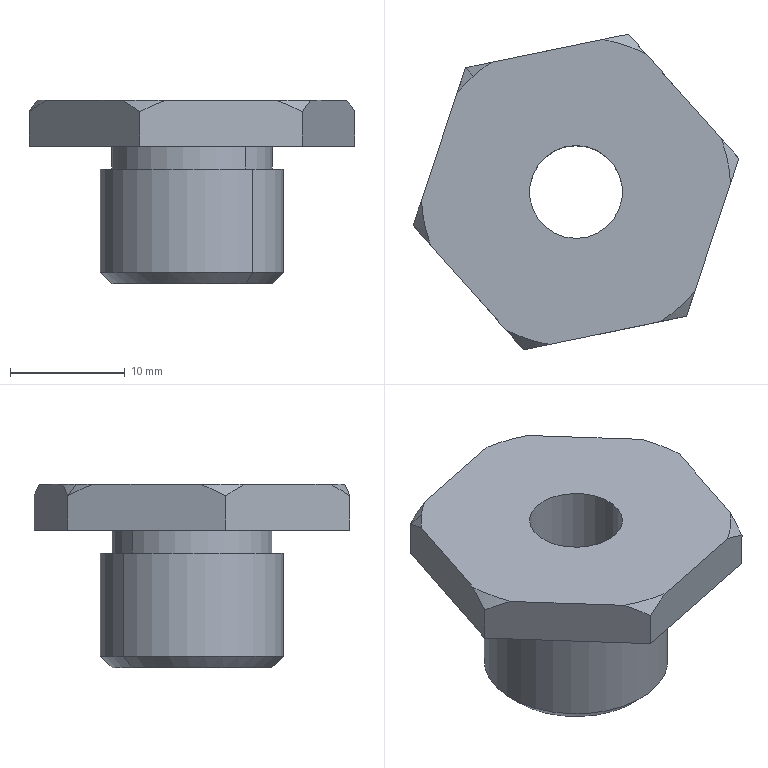Component | SolidWorks | DZ.KX.203-TC1505-20-18-05-93-1 | 1 solid | 25 faces | box 28.4 x 27.52 x 16 mm | volume 3651 mm3 | plane 10 | cone 9 | cylinder 6 | commonest cylinder face diameters 8.1 x2 16 x2 14 x2 | material Plain Carbon Steel
STEP:
#1=COLOUR_RGB('',0.7922,0.8196,0.9333);
#2=FILL_AREA_STYLE_COLOUR('',#1);
#3=FILL_AREA_STYLE('',(#2));
#4=SURFACE_STYLE_FILL_AREA(#3);
#5=SURFACE_SIDE_STYLE('',(#4));
#6=SURFACE_STYLE_USAGE(.BOTH.,#5);
#7=PRESENTATION_STYLE_ASSIGNMENT((#6));
#8=CARTESIAN_POINT('',(11.451,-31.991,4.057));
#9=VERTEX_POINT('',#8);
#10=CARTESIAN_POINT('',(11.817,-32.403,4.057));
#11=VERTEX_POINT('',#10);
#12=CARTESIAN_POINT('',(11.634,-32.197,4.057));
#13=DIRECTION('',(0.,-0.,-1.));
#14=DIRECTION('',(-0.6644,0.7474,-0.));
#15=AXIS2_PLACEMENT_3D('',#12,#13,#14);
#16=CIRCLE('',#15,0.2756);
#17=EDGE_CURVE('',#9,#11,#16,.T.);
#18=ORIENTED_EDGE('',*,*,#17,.F.);
#19=CARTESIAN_POINT('',(11.425,-31.962,4.097));
#20=VERTEX_POINT('',#19);
#21=CARTESIAN_POINT('',(11.451,-31.991,4.057));
#22=DIRECTION('',(-0.4698,0.5285,0.7071));
#23=VECTOR('',#22,39.37);
#24=LINE('',#21,#23);
#25=EDGE_CURVE('',#9,#20,#24,.T.);
#26=ORIENTED_EDGE('',*,*,#25,.T.);
#27=CARTESIAN_POINT('',(11.843,-32.433,4.097));
#28=VERTEX_POINT('',#27);
#29=CARTESIAN_POINT('',(11.634,-32.197,4.097));
#30=DIRECTION('',(-0.,0.,1.));
#31=DIRECTION('',(-0.6644,0.7474,-0.));
#32=AXIS2_PLACEMENT_3D('',#29,#30,#31);
#33=CIRCLE('',#32,0.315);
#34=EDGE_CURVE('',#28,#20,#33,.T.);
#35=ORIENTED_EDGE('',*,*,#34,.F.);
#36=CARTESIAN_POINT('',(11.817,-32.403,4.057));
#37=DIRECTION('',(0.4698,-0.5285,0.7071));
#38=VECTOR('',#37,39.37);
#39=LINE('',#36,#38);
#40=EDGE_CURVE('',#11,#28,#39,.T.);
#41=ORIENTED_EDGE('',*,*,#40,.F.);
#42=EDGE_LOOP('',(#18,#26,#35,#41));
#43=FACE_OUTER_BOUND('',#42,.T.);
#44=CARTESIAN_POINT('',(11.634,-32.197,4.057));
#45=DIRECTION('',(-0.,0.,1.));
#46=DIRECTION('',(0.6644,-0.7474,0.));
#47=AXIS2_PLACEMENT_3D('',#44,#45,#46);
#48=CONICAL_SURFACE('',#47,0.2756,0.7854);
#49=ADVANCED_FACE('',(#43),#48,.T.);
#50=CARTESIAN_POINT('',(11.528,-32.078,4.057));
#51=VERTEX_POINT('',#50);
#52=CARTESIAN_POINT('',(11.74,-32.316,4.057));
#53=VERTEX_POINT('',#52);
#54=CARTESIAN_POINT('',(11.634,-32.197,4.057));
#55=DIRECTION('',(-0.,0.,1.));
#56=DIRECTION('',(0.6644,-0.7474,0.));
#57=AXIS2_PLACEMENT_3D('',#54,#55,#56);
#58=CIRCLE('',#57,0.1594);
#59=EDGE_CURVE('',#51,#53,#58,.T.);
#60=ORIENTED_EDGE('',*,*,#59,.F.);
#61=CARTESIAN_POINT('',(11.528,-32.078,4.687));
#62=VERTEX_POINT('',#61);
#63=CARTESIAN_POINT('',(11.528,-32.078,4.687));
#64=DIRECTION('',(-0.,0.,1.));
#65=VECTOR('',#64,39.37);
#66=LINE('',#63,#65);
#67=EDGE_CURVE('',#51,#62,#66,.T.);
#68=ORIENTED_EDGE('',*,*,#67,.T.);
#69=CARTESIAN_POINT('',(11.74,-32.316,4.687));
#70=VERTEX_POINT('',#69);
#71=CARTESIAN_POINT('',(11.634,-32.197,4.687));
#72=DIRECTION('',(-0.,0.,1.));
#73=DIRECTION('',(0.6644,-0.7474,0.));
#74=AXIS2_PLACEMENT_3D('',#71,#72,#73);
#75=CIRCLE('',#74,0.1594);
#76=EDGE_CURVE('',#62,#70,#75,.T.);
#77=ORIENTED_EDGE('',*,*,#76,.T.);
#78=CARTESIAN_POINT('',(11.74,-32.316,4.687));
#79=DIRECTION('',(-0.,0.,1.));
#80=VECTOR('',#79,39.37);
#81=LINE('',#78,#80);
#82=EDGE_CURVE('',#53,#70,#81,.T.);
#83=ORIENTED_EDGE('',*,*,#82,.F.);
#84=EDGE_LOOP('',(#60,#68,#77,#83));
#85=FACE_OUTER_BOUND('',#84,.T.);
#86=CARTESIAN_POINT('',(11.634,-32.197,4.687));
#87=DIRECTION('',(-0.,0.,1.));
#88=DIRECTION('',(0.6644,-0.7474,0.));
#89=AXIS2_PLACEMENT_3D('',#86,#87,#88);
#90=CYLINDRICAL_SURFACE('',#89,0.1594);
#91=ADVANCED_FACE('',(#85),#90,.F.);
#92=CARTESIAN_POINT('',(11.281,-31.8,4.687));
#93=VERTEX_POINT('',#92);
#94=CARTESIAN_POINT('',(11.226,-31.856,4.687));
#95=VERTEX_POINT('',#94);
#96=CARTESIAN_POINT('',(11.634,-32.197,4.687));
#97=DIRECTION('',(-0.,0.,1.));
#98=DIRECTION('',(-0.6644,0.7474,-0.));
#99=AXIS2_PLACEMENT_3D('',#96,#97,#98);
#100=CIRCLE('',#99,0.5315);
#101=EDGE_CURVE('',#93,#95,#100,.T.);
#102=ORIENTED_EDGE('',*,*,#101,.F.);
#103=CARTESIAN_POINT('',(11.255,-31.77,4.648));
#104=VERTEX_POINT('',#103);
#105=CARTESIAN_POINT('',(11.255,-31.77,4.648));
#106=DIRECTION('',(-0.4698,0.5285,-0.7071));
#107=VECTOR('',#106,39.37);
#108=LINE('',#105,#107);
#109=EDGE_CURVE('',#93,#104,#108,.T.);
#110=ORIENTED_EDGE('',*,*,#109,.T.);
#111=CARTESIAN_POINT('',(11.226,-31.856,4.687));
#112=CARTESIAN_POINT('',(11.231,-31.842,4.682));
#113=CARTESIAN_POINT('',(11.236,-31.827,4.675));
#114=CARTESIAN_POINT('',(11.245,-31.798,4.662));
#115=CARTESIAN_POINT('',(11.25,-31.784,4.655));
#116=CARTESIAN_POINT('',(11.255,-31.77,4.648));
#117=B_SPLINE_CURVE_WITH_KNOTS('',3,(#111,#112,#113,#114,#115,#116),.UNSPECIFIED.,.F.,.F.,(4,2,4),(0.02484,0.02609,0.02734),.UNSPECIFIED.);
#118=EDGE_CURVE('',#95,#104,#117,.T.);
#119=ORIENTED_EDGE('',*,*,#118,.F.);
#120=EDGE_LOOP('',(#102,#110,#119));
#121=FACE_OUTER_BOUND('',#120,.T.);
#122=CARTESIAN_POINT('',(11.634,-32.197,4.648));
#123=DIRECTION('',(0.,-0.,-1.));
#124=DIRECTION('',(-0.6644,0.7474,-0.));
#125=AXIS2_PLACEMENT_3D('',#122,#123,#124);
#126=CONICAL_SURFACE('',#125,0.5709,0.7854);
#127=ADVANCED_FACE('',(#121),#126,.T.);
#128=ORIENTED_EDGE('',*,*,#34,.T.);
#129=CARTESIAN_POINT('',(11.425,-31.962,4.451));
#130=VERTEX_POINT('',#129);
#131=CARTESIAN_POINT('',(11.425,-31.962,4.057));
#132=DIRECTION('',(-0.,0.,1.));
#133=VECTOR('',#132,39.37);
#134=LINE('',#131,#133);
#135=EDGE_CURVE('',#20,#130,#134,.T.);
#136=ORIENTED_EDGE('',*,*,#135,.T.);
#137=CARTESIAN_POINT('',(11.843,-32.433,4.451));
#138=VERTEX_POINT('',#137);
#139=CARTESIAN_POINT('',(11.634,-32.197,4.451));
#140=DIRECTION('',(0.,-0.,-1.));
#141=DIRECTION('',(-0.6644,0.7474,-0.));
#142=AXIS2_PLACEMENT_3D('',#139,#140,#141);
#143=CIRCLE('',#142,0.315);
#144=EDGE_CURVE('',#130,#138,#143,.T.);
#145=ORIENTED_EDGE('',*,*,#144,.T.);
#146=CARTESIAN_POINT('',(11.843,-32.433,4.057));
#147=DIRECTION('',(-0.,0.,1.));
#148=VECTOR('',#147,39.37);
#149=LINE('',#146,#148);
#150=EDGE_CURVE('',#28,#138,#149,.T.);
#151=ORIENTED_EDGE('',*,*,#150,.F.);
#152=EDGE_LOOP('',(#128,#136,#145,#151));
#153=FACE_OUTER_BOUND('',#152,.T.);
#154=CARTESIAN_POINT('',(11.634,-32.197,4.057));
#155=DIRECTION('',(-0.,0.,1.));
#156=DIRECTION('',(0.6644,-0.7474,0.));
#157=AXIS2_PLACEMENT_3D('',#154,#155,#156);
#158=CYLINDRICAL_SURFACE('',#157,0.315);
#159=ADVANCED_FACE('',(#153),#158,.T.);
#160=CARTESIAN_POINT('',(11.451,-31.991,4.451));
#161=VERTEX_POINT('',#160);
#162=CARTESIAN_POINT('',(11.817,-32.403,4.451));
#163=VERTEX_POINT('',#162);
#164=CARTESIAN_POINT('',(11.634,-32.197,4.451));
#165=DIRECTION('',(0.,-0.,-1.));
#166=DIRECTION('',(-0.6644,0.7474,-0.));
#167=AXIS2_PLACEMENT_3D('',#164,#165,#166);
#168=CIRCLE('',#167,0.2756);
#169=EDGE_CURVE('',#161,#163,#168,.T.);
#170=ORIENTED_EDGE('',*,*,#169,.F.);
#171=CARTESIAN_POINT('',(11.451,-31.991,4.53));
#172=VERTEX_POINT('',#171);
#173=CARTESIAN_POINT('',(11.451,-31.991,4.451));
#174=DIRECTION('',(-0.,0.,1.));
#175=VECTOR('',#174,39.37);
#176=LINE('',#173,#175);
#177=EDGE_CURVE('',#161,#172,#176,.T.);
#178=ORIENTED_EDGE('',*,*,#177,.T.);
#179=CARTESIAN_POINT('',(11.817,-32.403,4.53));
#180=VERTEX_POINT('',#179);
#181=CARTESIAN_POINT('',(11.634,-32.197,4.53));
#182=DIRECTION('',(0.,-0.,-1.));
#183=DIRECTION('',(-0.6644,0.7474,-0.));
#184=AXIS2_PLACEMENT_3D('',#181,#182,#183);
#185=CIRCLE('',#184,0.2756);
#186=EDGE_CURVE('',#172,#180,#185,.T.);
#187=ORIENTED_EDGE('',*,*,#186,.T.);
#188=CARTESIAN_POINT('',(11.817,-32.403,4.451));
#189=DIRECTION('',(-0.,0.,1.));
#190=VECTOR('',#189,39.37);
#191=LINE('',#188,#190);
#192=EDGE_CURVE('',#163,#180,#191,.T.);
#193=ORIENTED_EDGE('',*,*,#192,.F.);
#194=EDGE_LOOP('',(#170,#178,#187,#193));
#195=FACE_OUTER_BOUND('',#194,.T.);
#196=CARTESIAN_POINT('',(11.634,-32.197,4.451));
#197=DIRECTION('',(-0.,0.,1.));
#198=DIRECTION('',(0.6644,-0.7474,0.));
#199=AXIS2_PLACEMENT_3D('',#196,#197,#198);
#200=CYLINDRICAL_SURFACE('',#199,0.2756);
#201=ADVANCED_FACE('',(#195),#200,.T.);
#202=CARTESIAN_POINT('',(12.193,-32.082,4.53));
#203=VERTEX_POINT('',#202);
#204=CARTESIAN_POINT('',(12.013,-32.624,4.53));
#205=VERTEX_POINT('',#204);
#206=CARTESIAN_POINT('',(12.193,-32.082,4.53));
#207=DIRECTION('',(-0.315,-0.9491,0.));
#208=VECTOR('',#207,39.37);
#209=LINE('',#206,#208);
#210=EDGE_CURVE('',#203,#205,#209,.T.);
#211=ORIENTED_EDGE('',*,*,#210,.T.);
#212=CARTESIAN_POINT('',(11.454,-32.739,4.53));
#213=VERTEX_POINT('',#212);
#214=CARTESIAN_POINT('',(12.013,-32.624,4.53));
#215=DIRECTION('',(-0.9794,-0.2017,0.));
#216=VECTOR('',#215,39.37);
#217=LINE('',#214,#216);
#218=EDGE_CURVE('',#205,#213,#217,.T.);
#219=ORIENTED_EDGE('',*,*,#218,.T.);
#220=CARTESIAN_POINT('',(11.075,-32.312,4.53));
#221=VERTEX_POINT('',#220);
#222=CARTESIAN_POINT('',(11.454,-32.739,4.53));
#223=DIRECTION('',(-0.6644,0.7474,-0.));
#224=VECTOR('',#223,39.37);
#225=LINE('',#222,#224);
#226=EDGE_CURVE('',#213,#221,#225,.T.);
#227=ORIENTED_EDGE('',*,*,#226,.T.);
#228=CARTESIAN_POINT('',(11.255,-31.77,4.53));
#229=VERTEX_POINT('',#228);
#230=CARTESIAN_POINT('',(11.075,-32.312,4.53));
#231=DIRECTION('',(0.315,0.9491,-0.));
#232=VECTOR('',#231,39.37);
#233=LINE('',#230,#232);
#234=EDGE_CURVE('',#221,#229,#233,.T.);
#235=ORIENTED_EDGE('',*,*,#234,.T.);
#236=CARTESIAN_POINT('',(11.814,-31.655,4.53));
#237=VERTEX_POINT('',#236);
#238=CARTESIAN_POINT('',(11.255,-31.77,4.53));
#239=DIRECTION('',(0.9794,0.2017,-0.));
#240=VECTOR('',#239,39.37);
#241=LINE('',#238,#240);
#242=EDGE_CURVE('',#229,#237,#241,.T.);
#243=ORIENTED_EDGE('',*,*,#242,.T.);
#244=CARTESIAN_POINT('',(11.814,-31.655,4.53));
#245=DIRECTION('',(0.6644,-0.7474,0.));
#246=VECTOR('',#245,39.37);
#247=LINE('',#244,#246);
#248=EDGE_CURVE('',#237,#203,#247,.T.);
#249=ORIENTED_EDGE('',*,*,#248,.T.);
#250=EDGE_LOOP('',(#211,#219,#227,#235,#243,#249));
#251=FACE_OUTER_BOUND('',#250,.T.);
#252=CARTESIAN_POINT('',(11.634,-32.197,4.53));
#253=DIRECTION('',(0.,-0.,-1.));
#254=DIRECTION('',(-0.6644,0.7474,-0.));
#255=AXIS2_PLACEMENT_3D('',#252,#253,#254);
#256=CIRCLE('',#255,0.2756);
#257=EDGE_CURVE('',#180,#172,#256,.T.);
#258=ORIENTED_EDGE('',*,*,#257,.F.);
#259=ORIENTED_EDGE('',*,*,#186,.F.);
#260=EDGE_LOOP('',(#258,#259));
#261=FACE_BOUND('',#260,.T.);
#262=CARTESIAN_POINT('',(11.634,-32.197,4.53));
#263=DIRECTION('',(0.,-0.,-1.));
#264=DIRECTION('',(-0.6644,0.7474,-0.));
#265=AXIS2_PLACEMENT_3D('',#262,#263,#264);
#266=PLANE('',#265);
#267=ADVANCED_FACE('',(#251,#261),#266,.T.);
#268=CARTESIAN_POINT('',(12.193,-32.082,4.648));
#269=VERTEX_POINT('',#268);
#270=CARTESIAN_POINT('',(12.193,-32.082,4.53));
#271=DIRECTION('',(-0.,0.,1.));
#272=VECTOR('',#271,39.37);
#273=LINE('',#270,#272);
#274=EDGE_CURVE('',#203,#269,#273,.T.);
#275=ORIENTED_EDGE('',*,*,#274,.T.);
#276=CARTESIAN_POINT('',(12.165,-32.168,4.687));
#277=VERTEX_POINT('',#276);
#278=CARTESIAN_POINT('',(12.193,-32.082,4.648));
#279=CARTESIAN_POINT('',(12.184,-32.11,4.663));
#280=CARTESIAN_POINT('',(12.174,-32.138,4.676));
#281=CARTESIAN_POINT('',(12.165,-32.168,4.687));
#282=B_SPLINE_CURVE_WITH_KNOTS('',3,(#278,#279,#280,#281),.UNSPECIFIED.,.F.,.F.,(4,4),(0.01221,0.01471),.UNSPECIFIED.);
#283=EDGE_CURVE('',#269,#277,#282,.T.);
#284=ORIENTED_EDGE('',*,*,#283,.T.);
#285=CARTESIAN_POINT('',(12.042,-32.538,4.687));
#286=VERTEX_POINT('',#285);
#287=CARTESIAN_POINT('',(12.193,-32.082,4.687));
#288=DIRECTION('',(-0.315,-0.9491,0.));
#289=VECTOR('',#288,39.37);
#290=LINE('',#287,#289);
#291=EDGE_CURVE('',#277,#286,#290,.T.);
#292=ORIENTED_EDGE('',*,*,#291,.T.);
#293=CARTESIAN_POINT('',(12.013,-32.624,4.648));
#294=VERTEX_POINT('',#293);
#295=CARTESIAN_POINT('',(12.042,-32.538,4.687));
#296=CARTESIAN_POINT('',(12.037,-32.553,4.682));
#297=CARTESIAN_POINT('',(12.032,-32.567,4.675));
#298=CARTESIAN_POINT('',(12.022,-32.596,4.662));
#299=CARTESIAN_POINT('',(12.018,-32.61,4.655));
#300=CARTESIAN_POINT('',(12.013,-32.624,4.648));
#301=B_SPLINE_CURVE_WITH_KNOTS('',3,(#295,#296,#297,#298,#299,#300),.UNSPECIFIED.,.F.,.F.,(4,2,4),(0.02484,0.02609,0.02734),.UNSPECIFIED.);
#302=EDGE_CURVE('',#286,#294,#301,.T.);
#303=ORIENTED_EDGE('',*,*,#302,.T.);
#304=CARTESIAN_POINT('',(12.013,-32.624,4.53));
#305=DIRECTION('',(-0.,0.,1.));
#306=VECTOR('',#305,39.37);
#307=LINE('',#304,#306);
#308=EDGE_CURVE('',#205,#294,#307,.T.);
#309=ORIENTED_EDGE('',*,*,#308,.F.);
#310=ORIENTED_EDGE('',*,*,#210,.F.);
#311=EDGE_LOOP('',(#275,#284,#292,#303,#309,#310));
#312=FACE_OUTER_BOUND('',#311,.T.);
#313=CARTESIAN_POINT('',(12.193,-32.082,4.53));
#314=DIRECTION('',(-0.9491,0.315,-0.));
#315=DIRECTION('',(0.315,0.9491,-0.));
#316=AXIS2_PLACEMENT_3D('',#313,#314,#315);
#317=PLANE('',#316);
#318=ADVANCED_FACE('',(#312),#317,.F.);
#319=ORIENTED_EDGE('',*,*,#308,.T.);
#320=CARTESIAN_POINT('',(11.925,-32.642,4.687));
#321=VERTEX_POINT('',#320);
#322=CARTESIAN_POINT('',(12.013,-32.624,4.648));
#323=CARTESIAN_POINT('',(11.984,-32.63,4.663));
#324=CARTESIAN_POINT('',(11.955,-32.636,4.676));
#325=CARTESIAN_POINT('',(11.925,-32.642,4.687));
#326=B_SPLINE_CURVE_WITH_KNOTS('',3,(#322,#323,#324,#325),.UNSPECIFIED.,.F.,.F.,(4,4),(0.01221,0.01471),.UNSPECIFIED.);
#327=EDGE_CURVE('',#294,#321,#326,.T.);
#328=ORIENTED_EDGE('',*,*,#327,.T.);
#329=CARTESIAN_POINT('',(11.542,-32.721,4.687));
#330=VERTEX_POINT('',#329);
#331=CARTESIAN_POINT('',(12.013,-32.624,4.687));
#332=DIRECTION('',(-0.9794,-0.2017,0.));
#333=VECTOR('',#332,39.37);
#334=LINE('',#331,#333);
#335=EDGE_CURVE('',#321,#330,#334,.T.);
#336=ORIENTED_EDGE('',*,*,#335,.T.);
#337=CARTESIAN_POINT('',(11.454,-32.739,4.648));
#338=VERTEX_POINT('',#337);
#339=CARTESIAN_POINT('',(11.542,-32.721,4.687));
#340=CARTESIAN_POINT('',(11.527,-32.724,4.682));
#341=CARTESIAN_POINT('',(11.512,-32.727,4.675));
#342=CARTESIAN_POINT('',(11.483,-32.733,4.662));
#343=CARTESIAN_POINT('',(11.468,-32.736,4.655));
#344=CARTESIAN_POINT('',(11.454,-32.739,4.648));
#345=B_SPLINE_CURVE_WITH_KNOTS('',3,(#339,#340,#341,#342,#343,#344),.UNSPECIFIED.,.F.,.F.,(4,2,4),(0.02484,0.02609,0.02734),.UNSPECIFIED.);
#346=EDGE_CURVE('',#330,#338,#345,.T.);
#347=ORIENTED_EDGE('',*,*,#346,.T.);
#348=CARTESIAN_POINT('',(11.454,-32.739,4.53));
#349=DIRECTION('',(-0.,0.,1.));
#350=VECTOR('',#349,39.37);
#351=LINE('',#348,#350);
#352=EDGE_CURVE('',#213,#338,#351,.T.);
#353=ORIENTED_EDGE('',*,*,#352,.F.);
#354=ORIENTED_EDGE('',*,*,#218,.F.);
#355=EDGE_LOOP('',(#319,#328,#336,#347,#353,#354));
#356=FACE_OUTER_BOUND('',#355,.T.);
#357=CARTESIAN_POINT('',(12.013,-32.624,4.53));
#358=DIRECTION('',(-0.2017,0.9794,-0.));
#359=DIRECTION('',(0.9794,0.2017,-0.));
#360=AXIS2_PLACEMENT_3D('',#357,#358,#359);
#361=PLANE('',#360);
#362=ADVANCED_FACE('',(#356),#361,.F.);
#363=ORIENTED_EDGE('',*,*,#352,.T.);
#364=CARTESIAN_POINT('',(11.394,-32.671,4.687));
#365=VERTEX_POINT('',#364);
#366=CARTESIAN_POINT('',(11.454,-32.739,4.648));
#367=CARTESIAN_POINT('',(11.435,-32.717,4.663));
#368=CARTESIAN_POINT('',(11.414,-32.694,4.676));
#369=CARTESIAN_POINT('',(11.394,-32.671,4.687));
#370=B_SPLINE_CURVE_WITH_KNOTS('',3,(#366,#367,#368,#369),.UNSPECIFIED.,.F.,.F.,(4,4),(0.01048,0.01297),.UNSPECIFIED.);
#371=EDGE_CURVE('',#338,#365,#370,.T.);
#372=ORIENTED_EDGE('',*,*,#371,.T.);
#373=CARTESIAN_POINT('',(11.135,-32.38,4.687));
#374=VERTEX_POINT('',#373);
#375=CARTESIAN_POINT('',(11.454,-32.739,4.687));
#376=DIRECTION('',(-0.6644,0.7474,-0.));
#377=VECTOR('',#376,39.37);
#378=LINE('',#375,#377);
#379=EDGE_CURVE('',#365,#374,#378,.T.);
#380=ORIENTED_EDGE('',*,*,#379,.T.);
#381=CARTESIAN_POINT('',(11.075,-32.312,4.648));
#382=VERTEX_POINT('',#381);
#383=CARTESIAN_POINT('',(11.135,-32.38,4.687));
#384=CARTESIAN_POINT('',(11.114,-32.357,4.676));
#385=CARTESIAN_POINT('',(11.094,-32.334,4.663));
#386=CARTESIAN_POINT('',(11.075,-32.312,4.648));
#387=B_SPLINE_CURVE_WITH_KNOTS('',3,(#383,#384,#385,#386),.UNSPECIFIED.,.F.,.F.,(4,4),(0.02308,0.02558),.UNSPECIFIED.);
#388=EDGE_CURVE('',#374,#382,#387,.T.);
#389=ORIENTED_EDGE('',*,*,#388,.T.);
#390=CARTESIAN_POINT('',(11.075,-32.312,4.53));
#391=DIRECTION('',(-0.,0.,1.));
#392=VECTOR('',#391,39.37);
#393=LINE('',#390,#392);
#394=EDGE_CURVE('',#221,#382,#393,.T.);
#395=ORIENTED_EDGE('',*,*,#394,.F.);
#396=ORIENTED_EDGE('',*,*,#226,.F.);
#397=EDGE_LOOP('',(#363,#372,#380,#389,#395,#396));
#398=FACE_OUTER_BOUND('',#397,.T.);
#399=CARTESIAN_POINT('',(11.454,-32.739,4.53));
#400=DIRECTION('',(0.7474,0.6644,-0.));
#401=DIRECTION('',(0.6644,-0.7474,0.));
#402=AXIS2_PLACEMENT_3D('',#399,#400,#401);
#403=PLANE('',#402);
#404=ADVANCED_FACE('',(#398),#403,.F.);
#405=ORIENTED_EDGE('',*,*,#394,.T.);
#406=CARTESIAN_POINT('',(11.103,-32.227,4.687));
#407=VERTEX_POINT('',#406);
#408=CARTESIAN_POINT('',(11.075,-32.312,4.648));
#409=CARTESIAN_POINT('',(11.084,-32.284,4.663));
#410=CARTESIAN_POINT('',(11.093,-32.256,4.676));
#411=CARTESIAN_POINT('',(11.103,-32.227,4.687));
#412=B_SPLINE_CURVE_WITH_KNOTS('',3,(#408,#409,#410,#411),.UNSPECIFIED.,.F.,.F.,(4,4),(0.01221,0.01471),.UNSPECIFIED.);
#413=EDGE_CURVE('',#382,#407,#412,.T.);
#414=ORIENTED_EDGE('',*,*,#413,.T.);
#415=CARTESIAN_POINT('',(11.075,-32.312,4.687));
#416=DIRECTION('',(0.315,0.9491,-0.));
#417=VECTOR('',#416,39.37);
#418=LINE('',#415,#417);
#419=EDGE_CURVE('',#407,#95,#418,.T.);
#420=ORIENTED_EDGE('',*,*,#419,.T.);
#421=ORIENTED_EDGE('',*,*,#118,.T.);
#422=CARTESIAN_POINT('',(11.255,-31.77,4.53));
#423=DIRECTION('',(-0.,0.,1.));
#424=VECTOR('',#423,39.37);
#425=LINE('',#422,#424);
#426=EDGE_CURVE('',#229,#104,#425,.T.);
#427=ORIENTED_EDGE('',*,*,#426,.F.);
#428=ORIENTED_EDGE('',*,*,#234,.F.);
#429=EDGE_LOOP('',(#405,#414,#420,#421,#427,#428));
#430=FACE_OUTER_BOUND('',#429,.T.);
#431=CARTESIAN_POINT('',(11.075,-32.312,4.53));
#432=DIRECTION('',(0.9491,-0.315,0.));
#433=DIRECTION('',(-0.315,-0.9491,0.));
#434=AXIS2_PLACEMENT_3D('',#431,#432,#433);
#435=PLANE('',#434);
#436=ADVANCED_FACE('',(#430),#435,.F.);
#437=ORIENTED_EDGE('',*,*,#426,.T.);
#438=CARTESIAN_POINT('',(11.343,-31.752,4.687));
#439=VERTEX_POINT('',#438);
#440=CARTESIAN_POINT('',(11.255,-31.77,4.648));
#441=CARTESIAN_POINT('',(11.283,-31.765,4.663));
#442=CARTESIAN_POINT('',(11.313,-31.758,4.676));
#443=CARTESIAN_POINT('',(11.343,-31.752,4.687));
#444=B_SPLINE_CURVE_WITH_KNOTS('',3,(#440,#441,#442,#443),.UNSPECIFIED.,.F.,.F.,(4,4),(0.01221,0.01471),.UNSPECIFIED.);
#445=EDGE_CURVE('',#104,#439,#444,.T.);
#446=ORIENTED_EDGE('',*,*,#445,.T.);
#447=CARTESIAN_POINT('',(11.725,-31.674,4.687));
#448=VERTEX_POINT('',#447);
#449=CARTESIAN_POINT('',(11.255,-31.77,4.687));
#450=DIRECTION('',(0.9794,0.2017,-0.));
#451=VECTOR('',#450,39.37);
#452=LINE('',#449,#451);
#453=EDGE_CURVE('',#439,#448,#452,.T.);
#454=ORIENTED_EDGE('',*,*,#453,.T.);
#455=CARTESIAN_POINT('',(11.814,-31.655,4.648));
#456=VERTEX_POINT('',#455);
#457=CARTESIAN_POINT('',(11.725,-31.674,4.687));
#458=CARTESIAN_POINT('',(11.74,-31.67,4.682));
#459=CARTESIAN_POINT('',(11.755,-31.667,4.675));
#460=CARTESIAN_POINT('',(11.785,-31.661,4.662));
#461=CARTESIAN_POINT('',(11.799,-31.658,4.655));
#462=CARTESIAN_POINT('',(11.814,-31.655,4.648));
#463=B_SPLINE_CURVE_WITH_KNOTS('',3,(#457,#458,#459,#460,#461,#462),.UNSPECIFIED.,.F.,.F.,(4,2,4),(0.02484,0.02609,0.02734),.UNSPECIFIED.);
#464=EDGE_CURVE('',#448,#456,#463,.T.);
#465=ORIENTED_EDGE('',*,*,#464,.T.);
#466=CARTESIAN_POINT('',(11.814,-31.655,4.53));
#467=DIRECTION('',(-0.,0.,1.));
#468=VECTOR('',#467,39.37);
#469=LINE('',#466,#468);
#470=EDGE_CURVE('',#237,#456,#469,.T.);
#471=ORIENTED_EDGE('',*,*,#470,.F.);
#472=ORIENTED_EDGE('',*,*,#242,.F.);
#473=EDGE_LOOP('',(#437,#446,#454,#465,#471,#472));
#474=FACE_OUTER_BOUND('',#473,.T.);
#475=CARTESIAN_POINT('',(11.255,-31.77,4.53));
#476=DIRECTION('',(0.2017,-0.9794,0.));
#477=DIRECTION('',(-0.9794,-0.2017,0.));
#478=AXIS2_PLACEMENT_3D('',#475,#476,#477);
#479=PLANE('',#478);
#480=ADVANCED_FACE('',(#474),#479,.F.);
#481=ORIENTED_EDGE('',*,*,#470,.T.);
#482=CARTESIAN_POINT('',(11.874,-31.723,4.687));
#483=VERTEX_POINT('',#482);
#484=CARTESIAN_POINT('',(11.814,-31.655,4.648));
#485=CARTESIAN_POINT('',(11.833,-31.677,4.663));
#486=CARTESIAN_POINT('',(11.853,-31.7,4.676));
#487=CARTESIAN_POINT('',(11.874,-31.723,4.687));
#488=B_SPLINE_CURVE_WITH_KNOTS('',3,(#484,#485,#486,#487),.UNSPECIFIED.,.F.,.F.,(4,4),(0.01048,0.01297),.UNSPECIFIED.);
#489=EDGE_CURVE('',#456,#483,#488,.T.);
#490=ORIENTED_EDGE('',*,*,#489,.T.);
#491=CARTESIAN_POINT('',(12.133,-32.014,4.687));
#492=VERTEX_POINT('',#491);
#493=CARTESIAN_POINT('',(11.814,-31.655,4.687));
#494=DIRECTION('',(0.6644,-0.7474,0.));
#495=VECTOR('',#494,39.37);
#496=LINE('',#493,#495);
#497=EDGE_CURVE('',#483,#492,#496,.T.);
#498=ORIENTED_EDGE('',*,*,#497,.T.);
#499=CARTESIAN_POINT('',(12.133,-32.014,4.687));
#500=CARTESIAN_POINT('',(12.154,-32.038,4.676));
#501=CARTESIAN_POINT('',(12.173,-32.06,4.663));
#502=CARTESIAN_POINT('',(12.193,-32.082,4.648));
#503=B_SPLINE_CURVE_WITH_KNOTS('',3,(#499,#500,#501,#502),.UNSPECIFIED.,.F.,.F.,(4,4),(0.02308,0.02558),.UNSPECIFIED.);
#504=EDGE_CURVE('',#492,#269,#503,.T.);
#505=ORIENTED_EDGE('',*,*,#504,.T.);
#506=ORIENTED_EDGE('',*,*,#274,.F.);
#507=ORIENTED_EDGE('',*,*,#248,.F.);
#508=EDGE_LOOP('',(#481,#490,#498,#505,#506,#507));
#509=FACE_OUTER_BOUND('',#508,.T.);
#510=CARTESIAN_POINT('',(11.814,-31.655,4.53));
#511=DIRECTION('',(-0.7474,-0.6644,0.));
#512=DIRECTION('',(-0.6644,0.7474,-0.));
#513=AXIS2_PLACEMENT_3D('',#510,#511,#512);
#514=PLANE('',#513);
#515=ADVANCED_FACE('',(#509),#514,.F.);
#516=CARTESIAN_POINT('',(11.634,-32.197,4.687));
#517=DIRECTION('',(-0.,0.,1.));
#518=DIRECTION('',(0.6644,-0.7474,0.));
#519=AXIS2_PLACEMENT_3D('',#516,#517,#518);
#520=CIRCLE('',#519,0.1594);
#521=EDGE_CURVE('',#70,#62,#520,.T.);
#522=ORIENTED_EDGE('',*,*,#521,.F.);
#523=ORIENTED_EDGE('',*,*,#76,.F.);
#524=EDGE_LOOP('',(#522,#523));
#525=FACE_BOUND('',#524,.T.);
#526=ORIENTED_EDGE('',*,*,#419,.F.);
#527=CARTESIAN_POINT('',(11.634,-32.197,4.687));
#528=DIRECTION('',(-0.,0.,1.));
#529=DIRECTION('',(-0.6644,0.7474,-0.));
#530=AXIS2_PLACEMENT_3D('',#527,#528,#529);
#531=CIRCLE('',#530,0.5315);
#532=EDGE_CURVE('',#407,#374,#531,.T.);
#533=ORIENTED_EDGE('',*,*,#532,.T.);
#534=ORIENTED_EDGE('',*,*,#379,.F.);
#535=CARTESIAN_POINT('',(11.634,-32.197,4.687));
#536=DIRECTION('',(-0.,0.,1.));
#537=DIRECTION('',(-0.6644,0.7474,-0.));
#538=AXIS2_PLACEMENT_3D('',#535,#536,#537);
#539=CIRCLE('',#538,0.5315);
#540=EDGE_CURVE('',#365,#330,#539,.T.);
#541=ORIENTED_EDGE('',*,*,#540,.T.);
#542=ORIENTED_EDGE('',*,*,#335,.F.);
#543=CARTESIAN_POINT('',(11.634,-32.197,4.687));
#544=DIRECTION('',(-0.,0.,1.));
#545=DIRECTION('',(-0.6644,0.7474,-0.));
#546=AXIS2_PLACEMENT_3D('',#543,#544,#545);
#547=CIRCLE('',#546,0.5315);
#548=EDGE_CURVE('',#321,#286,#547,.T.);
#549=ORIENTED_EDGE('',*,*,#548,.T.);
#550=ORIENTED_EDGE('',*,*,#291,.F.);
#551=CARTESIAN_POINT('',(11.634,-32.197,4.687));
#552=DIRECTION('',(-0.,0.,1.));
#553=DIRECTION('',(-0.6644,0.7474,-0.));
#554=AXIS2_PLACEMENT_3D('',#551,#552,#553);
#555=CIRCLE('',#554,0.5315);
#556=EDGE_CURVE('',#277,#492,#555,.T.);
#557=ORIENTED_EDGE('',*,*,#556,.T.);
#558=ORIENTED_EDGE('',*,*,#497,.F.);
#559=CARTESIAN_POINT('',(11.634,-32.197,4.687));
#560=DIRECTION('',(-0.,0.,1.));
#561=DIRECTION('',(-0.6644,0.7474,-0.));
#562=AXIS2_PLACEMENT_3D('',#559,#560,#561);
#563=CIRCLE('',#562,0.5315);
#564=EDGE_CURVE('',#483,#448,#563,.T.);
#565=ORIENTED_EDGE('',*,*,#564,.T.);
#566=ORIENTED_EDGE('',*,*,#453,.F.);
#567=CARTESIAN_POINT('',(11.634,-32.197,4.687));
#568=DIRECTION('',(-0.,0.,1.));
#569=DIRECTION('',(-0.6644,0.7474,-0.));
#570=AXIS2_PLACEMENT_3D('',#567,#568,#569);
#571=CIRCLE('',#570,0.5315);
#572=EDGE_CURVE('',#439,#93,#571,.T.);
#573=ORIENTED_EDGE('',*,*,#572,.T.);
#574=ORIENTED_EDGE('',*,*,#101,.T.);
#575=EDGE_LOOP('',(#526,#533,#534,#541,#542,#549,#550,#557,#558,#565,#566,#573,#574));
#576=FACE_OUTER_BOUND('',#575,.T.);
#577=CARTESIAN_POINT('',(11.634,-32.197,4.687));
#578=DIRECTION('',(0.,-0.,-1.));
#579=DIRECTION('',(-0.6644,0.7474,-0.));
#580=AXIS2_PLACEMENT_3D('',#577,#578,#579);
#581=PLANE('',#580);
#582=ADVANCED_FACE('',(#525,#576),#581,.F.);
#583=ORIENTED_EDGE('',*,*,#177,.F.);
#584=CARTESIAN_POINT('',(11.634,-32.197,4.451));
#585=DIRECTION('',(0.,-0.,-1.));
#586=DIRECTION('',(-0.6644,0.7474,-0.));
#587=AXIS2_PLACEMENT_3D('',#584,#585,#586);
#588=CIRCLE('',#587,0.2756);
#589=EDGE_CURVE('',#163,#161,#588,.T.);
#590=ORIENTED_EDGE('',*,*,#589,.F.);
#591=ORIENTED_EDGE('',*,*,#192,.T.);
#592=ORIENTED_EDGE('',*,*,#257,.T.);
#593=EDGE_LOOP('',(#583,#590,#591,#592));
#594=FACE_OUTER_BOUND('',#593,.T.);
#595=CARTESIAN_POINT('',(11.634,-32.197,4.451));
#596=DIRECTION('',(-0.,0.,1.));
#597=DIRECTION('',(0.6644,-0.7474,0.));
#598=AXIS2_PLACEMENT_3D('',#595,#596,#597);
#599=CYLINDRICAL_SURFACE('',#598,0.2756);
#600=ADVANCED_FACE('',(#594),#599,.T.);
#601=CARTESIAN_POINT('',(11.634,-32.197,4.451));
#602=DIRECTION('',(0.,-0.,-1.));
#603=DIRECTION('',(-0.6644,0.7474,-0.));
#604=AXIS2_PLACEMENT_3D('',#601,#602,#603);
#605=CIRCLE('',#604,0.315);
#606=EDGE_CURVE('',#138,#130,#605,.T.);
#607=ORIENTED_EDGE('',*,*,#606,.F.);
#608=ORIENTED_EDGE('',*,*,#144,.F.);
#609=EDGE_LOOP('',(#607,#608));
#610=FACE_OUTER_BOUND('',#609,.T.);
#611=ORIENTED_EDGE('',*,*,#589,.T.);
#612=ORIENTED_EDGE('',*,*,#169,.T.);
#613=EDGE_LOOP('',(#611,#612));
#614=FACE_BOUND('',#613,.T.);
#615=CARTESIAN_POINT('',(11.634,-32.197,4.451));
#616=DIRECTION('',(0.,-0.,-1.));
#617=DIRECTION('',(-0.6644,0.7474,-0.));
#618=AXIS2_PLACEMENT_3D('',#615,#616,#617);
#619=PLANE('',#618);
#620=ADVANCED_FACE('',(#610,#614),#619,.F.);
#621=ORIENTED_EDGE('',*,*,#135,.F.);
#622=CARTESIAN_POINT('',(11.634,-32.197,4.097));
#623=DIRECTION('',(-0.,0.,1.));
#624=DIRECTION('',(-0.6644,0.7474,-0.));
#625=AXIS2_PLACEMENT_3D('',#622,#623,#624);
#626=CIRCLE('',#625,0.315);
#627=EDGE_CURVE('',#20,#28,#626,.T.);
#628=ORIENTED_EDGE('',*,*,#627,.T.);
#629=ORIENTED_EDGE('',*,*,#150,.T.);
#630=ORIENTED_EDGE('',*,*,#606,.T.);
#631=EDGE_LOOP('',(#621,#628,#629,#630));
#632=FACE_OUTER_BOUND('',#631,.T.);
#633=CARTESIAN_POINT('',(11.634,-32.197,4.057));
#634=DIRECTION('',(-0.,0.,1.));
#635=DIRECTION('',(0.6644,-0.7474,0.));
#636=AXIS2_PLACEMENT_3D('',#633,#634,#635);
#637=CYLINDRICAL_SURFACE('',#636,0.315);
#638=ADVANCED_FACE('',(#632),#637,.T.);
#639=CARTESIAN_POINT('',(11.634,-32.197,4.057));
#640=DIRECTION('',(0.,-0.,-1.));
#641=DIRECTION('',(-0.6644,0.7474,-0.));
#642=AXIS2_PLACEMENT_3D('',#639,#640,#641);
#643=CIRCLE('',#642,0.2756);
#644=EDGE_CURVE('',#11,#9,#643,.T.);
#645=ORIENTED_EDGE('',*,*,#644,.T.);
#646=ORIENTED_EDGE('',*,*,#17,.T.);
#647=EDGE_LOOP('',(#645,#646));
#648=FACE_OUTER_BOUND('',#647,.T.);
#649=CARTESIAN_POINT('',(11.634,-32.197,4.057));
#650=DIRECTION('',(-0.,0.,1.));
#651=DIRECTION('',(0.6644,-0.7474,0.));
#652=AXIS2_PLACEMENT_3D('',#649,#650,#651);
#653=CIRCLE('',#652,0.1594);
#654=EDGE_CURVE('',#53,#51,#653,.T.);
#655=ORIENTED_EDGE('',*,*,#654,.T.);
#656=ORIENTED_EDGE('',*,*,#59,.T.);
#657=EDGE_LOOP('',(#655,#656));
#658=FACE_BOUND('',#657,.T.);
#659=CARTESIAN_POINT('',(11.634,-32.197,4.057));
#660=DIRECTION('',(0.,-0.,-1.));
#661=DIRECTION('',(-0.6644,0.7474,-0.));
#662=AXIS2_PLACEMENT_3D('',#659,#660,#661);
#663=PLANE('',#662);
#664=ADVANCED_FACE('',(#648,#658),#663,.T.);
#665=ORIENTED_EDGE('',*,*,#109,.F.);
#666=ORIENTED_EDGE('',*,*,#572,.F.);
#667=ORIENTED_EDGE('',*,*,#445,.F.);
#668=EDGE_LOOP('',(#665,#666,#667));
#669=FACE_OUTER_BOUND('',#668,.T.);
#670=CARTESIAN_POINT('',(11.634,-32.197,4.648));
#671=DIRECTION('',(0.,-0.,-1.));
#672=DIRECTION('',(-0.6644,0.7474,-0.));
#673=AXIS2_PLACEMENT_3D('',#670,#671,#672);
#674=CONICAL_SURFACE('',#673,0.5709,0.7854);
#675=ADVANCED_FACE('',(#669),#674,.T.);
#676=ORIENTED_EDGE('',*,*,#564,.F.);
#677=ORIENTED_EDGE('',*,*,#489,.F.);
#678=ORIENTED_EDGE('',*,*,#464,.F.);
#679=EDGE_LOOP('',(#676,#677,#678));
#680=FACE_OUTER_BOUND('',#679,.T.);
#681=CARTESIAN_POINT('',(11.634,-32.197,4.648));
#682=DIRECTION('',(0.,-0.,-1.));
#683=DIRECTION('',(-0.6644,0.7474,-0.));
#684=AXIS2_PLACEMENT_3D('',#681,#682,#683);
#685=CONICAL_SURFACE('',#684,0.5709,0.7854);
#686=ADVANCED_FACE('',(#680),#685,.T.);
#687=ORIENTED_EDGE('',*,*,#504,.F.);
#688=ORIENTED_EDGE('',*,*,#556,.F.);
#689=ORIENTED_EDGE('',*,*,#283,.F.);
#690=EDGE_LOOP('',(#687,#688,#689));
#691=FACE_OUTER_BOUND('',#690,.T.);
#692=CARTESIAN_POINT('',(11.634,-32.197,4.648));
#693=DIRECTION('',(0.,-0.,-1.));
#694=DIRECTION('',(-0.6644,0.7474,-0.));
#695=AXIS2_PLACEMENT_3D('',#692,#693,#694);
#696=CONICAL_SURFACE('',#695,0.5709,0.7854);
#697=ADVANCED_FACE('',(#691),#696,.T.);
#698=ORIENTED_EDGE('',*,*,#548,.F.);
#699=ORIENTED_EDGE('',*,*,#327,.F.);
#700=ORIENTED_EDGE('',*,*,#302,.F.);
#701=EDGE_LOOP('',(#698,#699,#700));
#702=FACE_OUTER_BOUND('',#701,.T.);
#703=CARTESIAN_POINT('',(11.634,-32.197,4.648));
#704=DIRECTION('',(0.,-0.,-1.));
#705=DIRECTION('',(-0.6644,0.7474,-0.));
#706=AXIS2_PLACEMENT_3D('',#703,#704,#705);
#707=CONICAL_SURFACE('',#706,0.5709,0.7854);
#708=ADVANCED_FACE('',(#702),#707,.T.);
#709=ORIENTED_EDGE('',*,*,#540,.F.);
#710=ORIENTED_EDGE('',*,*,#371,.F.);
#711=ORIENTED_EDGE('',*,*,#346,.F.);
#712=EDGE_LOOP('',(#709,#710,#711));
#713=FACE_OUTER_BOUND('',#712,.T.);
#714=CARTESIAN_POINT('',(11.634,-32.197,4.648));
#715=DIRECTION('',(0.,-0.,-1.));
#716=DIRECTION('',(-0.6644,0.7474,-0.));
#717=AXIS2_PLACEMENT_3D('',#714,#715,#716);
#718=CONICAL_SURFACE('',#717,0.5709,0.7854);
#719=ADVANCED_FACE('',(#713),#718,.T.);
#720=ORIENTED_EDGE('',*,*,#532,.F.);
#721=ORIENTED_EDGE('',*,*,#413,.F.);
#722=ORIENTED_EDGE('',*,*,#388,.F.);
#723=EDGE_LOOP('',(#720,#721,#722));
#724=FACE_OUTER_BOUND('',#723,.T.);
#725=CARTESIAN_POINT('',(11.634,-32.197,4.648));
#726=DIRECTION('',(0.,-0.,-1.));
#727=DIRECTION('',(-0.6644,0.7474,-0.));
#728=AXIS2_PLACEMENT_3D('',#725,#726,#727);
#729=CONICAL_SURFACE('',#728,0.5709,0.7854);
#730=ADVANCED_FACE('',(#724),#729,.T.);
#731=ORIENTED_EDGE('',*,*,#67,.F.);
#732=ORIENTED_EDGE('',*,*,#654,.F.);
#733=ORIENTED_EDGE('',*,*,#82,.T.);
#734=ORIENTED_EDGE('',*,*,#521,.T.);
#735=EDGE_LOOP('',(#731,#732,#733,#734));
#736=FACE_OUTER_BOUND('',#735,.T.);
#737=CARTESIAN_POINT('',(11.634,-32.197,4.687));
#738=DIRECTION('',(-0.,0.,1.));
#739=DIRECTION('',(0.6644,-0.7474,0.));
#740=AXIS2_PLACEMENT_3D('',#737,#738,#739);
#741=CYLINDRICAL_SURFACE('',#740,0.1594);
#742=ADVANCED_FACE('',(#736),#741,.F.);
#743=ORIENTED_EDGE('',*,*,#25,.F.);
#744=ORIENTED_EDGE('',*,*,#644,.F.);
#745=ORIENTED_EDGE('',*,*,#40,.T.);
#746=ORIENTED_EDGE('',*,*,#627,.F.);
#747=EDGE_LOOP('',(#743,#744,#745,#746));
#748=FACE_OUTER_BOUND('',#747,.T.);
#749=CARTESIAN_POINT('',(11.634,-32.197,4.057));
#750=DIRECTION('',(-0.,0.,1.));
#751=DIRECTION('',(0.6644,-0.7474,0.));
#752=AXIS2_PLACEMENT_3D('',#749,#750,#751);
#753=CONICAL_SURFACE('',#752,0.2756,0.7854);
#754=ADVANCED_FACE('',(#748),#753,.T.);
#755=CLOSED_SHELL('',(#49,#91,#127,#159,#201,#267,#318,#362,#404,#436,#480,#515,#582,#600,#620,#638,#664,#675,#686,#697,#708,#719,#730,#742,#754));
#756=MANIFOLD_SOLID_BREP('',#755);
#757=STYLED_ITEM('',(#7),#756);
#758=PRESENTATION_LAYER_ASSIGNMENT('','',(#757));
#759=(LENGTH_UNIT()NAMED_UNIT(*)SI_UNIT($,.METRE.));
#760=LENGTH_MEASURE_WITH_UNIT(LENGTH_MEASURE(0.0254),#759);
#761=DIMENSIONAL_EXPONENTS(1.,0.,0.,0.,0.,0.,0.);
#762=(CONVERSION_BASED_UNIT('',#760)LENGTH_UNIT()NAMED_UNIT(#761));
#763=UNCERTAINTY_MEASURE_WITH_UNIT(LENGTH_MEASURE(0.00001),#762,'','');
#764=(NAMED_UNIT(*)PLANE_ANGLE_UNIT()SI_UNIT($,.RADIAN.));
#765=(NAMED_UNIT(*)SI_UNIT($,.STERADIAN.)SOLID_ANGLE_UNIT());
#766=(GEOMETRIC_REPRESENTATION_CONTEXT(3)GLOBAL_UNCERTAINTY_ASSIGNED_CONTEXT((#763))GLOBAL_UNIT_ASSIGNED_CONTEXT((#762,#764,#765))REPRESENTATION_CONTEXT('',''));
#767=MECHANICAL_DESIGN_GEOMETRIC_PRESENTATION_REPRESENTATION('',(#757),#766);
#768=CARTESIAN_POINT('',(0.,0.,0.));
#769=DIRECTION('',(0.,0.,1.));
#770=DIRECTION('',(1.,0.,0.));
#771=AXIS2_PLACEMENT_3D('',#768,#769,#770);
#772=(LENGTH_UNIT()NAMED_UNIT(*)SI_UNIT($,.METRE.));
#773=LENGTH_MEASURE_WITH_UNIT(LENGTH_MEASURE(0.0254),#772);
#774=DIMENSIONAL_EXPONENTS(1.,0.,0.,0.,0.,0.,0.);
#775=(CONVERSION_BASED_UNIT('',#773)LENGTH_UNIT()NAMED_UNIT(#774));
#776=UNCERTAINTY_MEASURE_WITH_UNIT(LENGTH_MEASURE(0.00001),#775,'','');
#777=(NAMED_UNIT(*)PLANE_ANGLE_UNIT()SI_UNIT($,.RADIAN.));
#778=(NAMED_UNIT(*)SI_UNIT($,.STERADIAN.)SOLID_ANGLE_UNIT());
#779=(GEOMETRIC_REPRESENTATION_CONTEXT(3)GLOBAL_UNCERTAINTY_ASSIGNED_CONTEXT((#776))GLOBAL_UNIT_ASSIGNED_CONTEXT((#775,#777,#778))REPRESENTATION_CONTEXT('',''));
#780=ADVANCED_BREP_SHAPE_REPRESENTATION('',(#756,#771),#779);